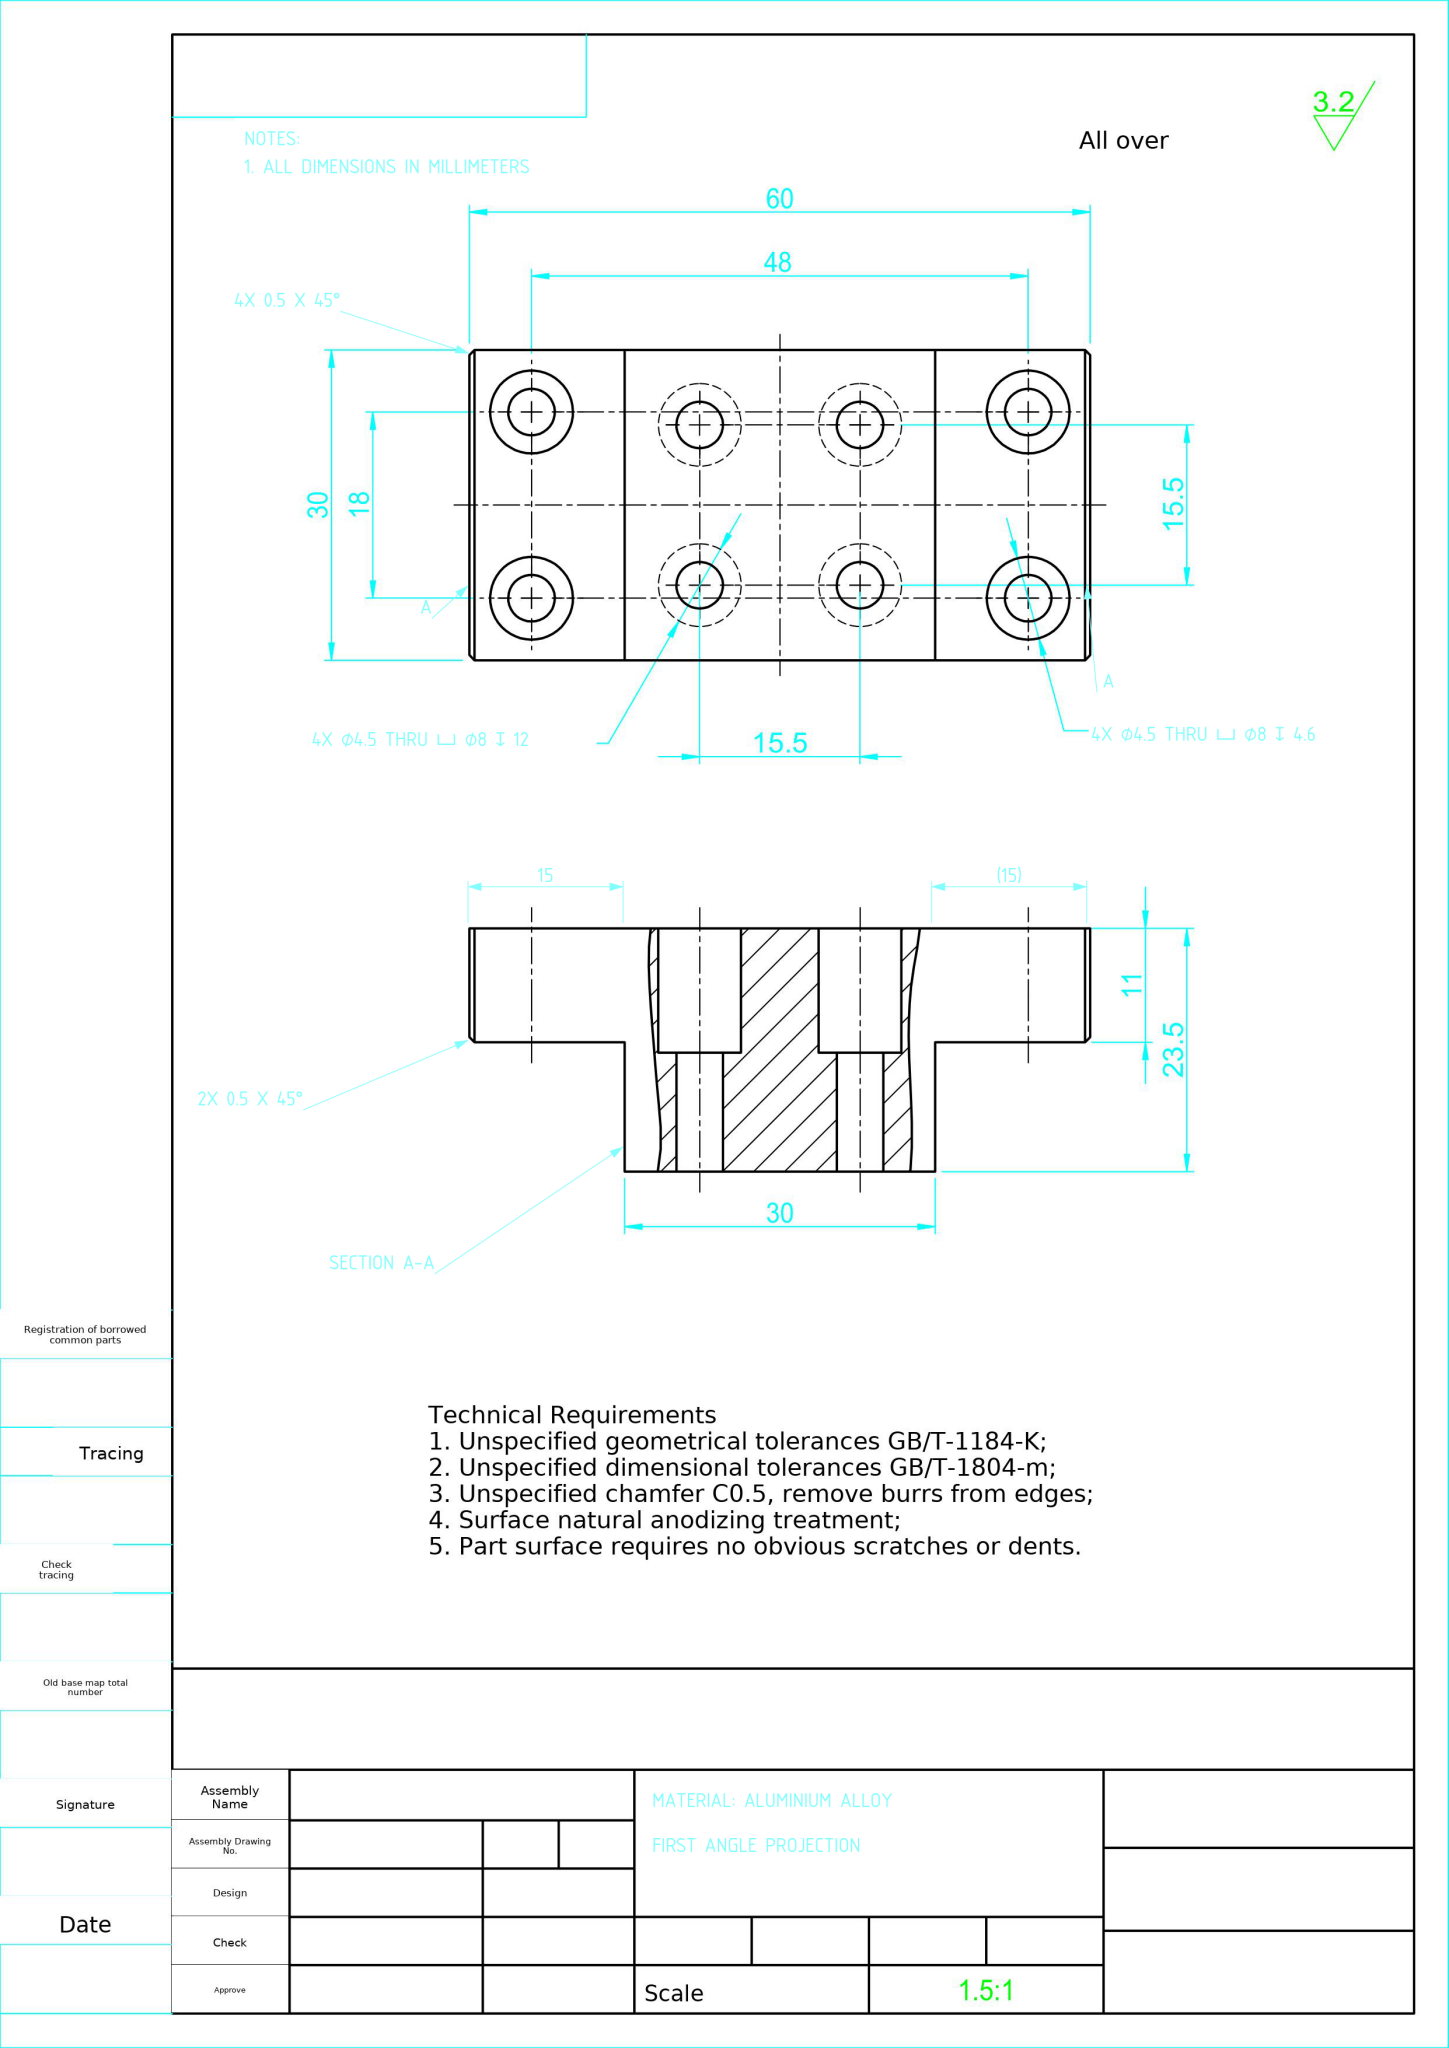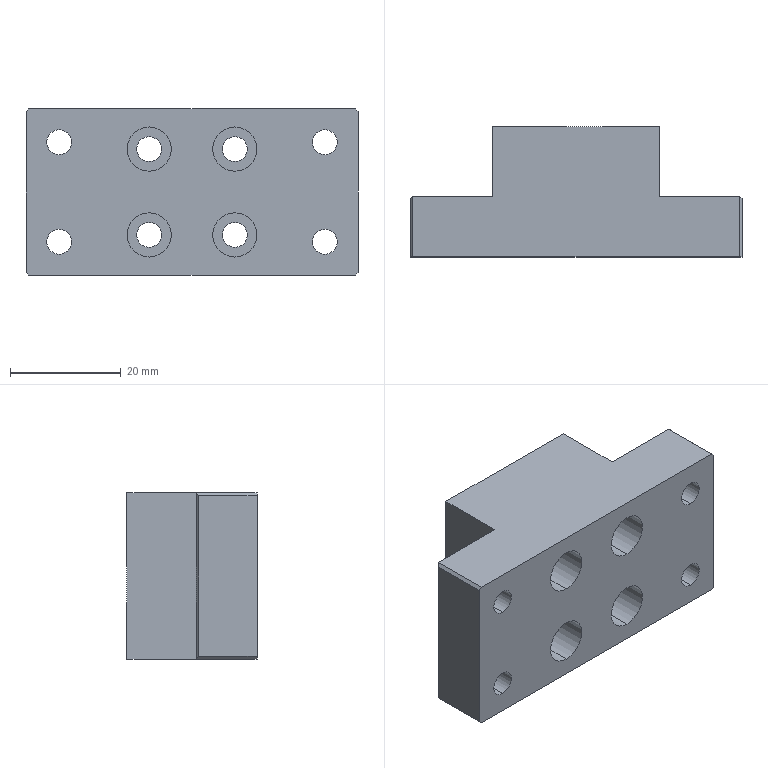Part | NX | mm | 1 solid | 56 faces | box 60 x 23.5 x 30 mm | volume 26561 mm3 | cylinder 32 | plane 24 | commonest cylinder face diameters 8 x16 4.5 x16